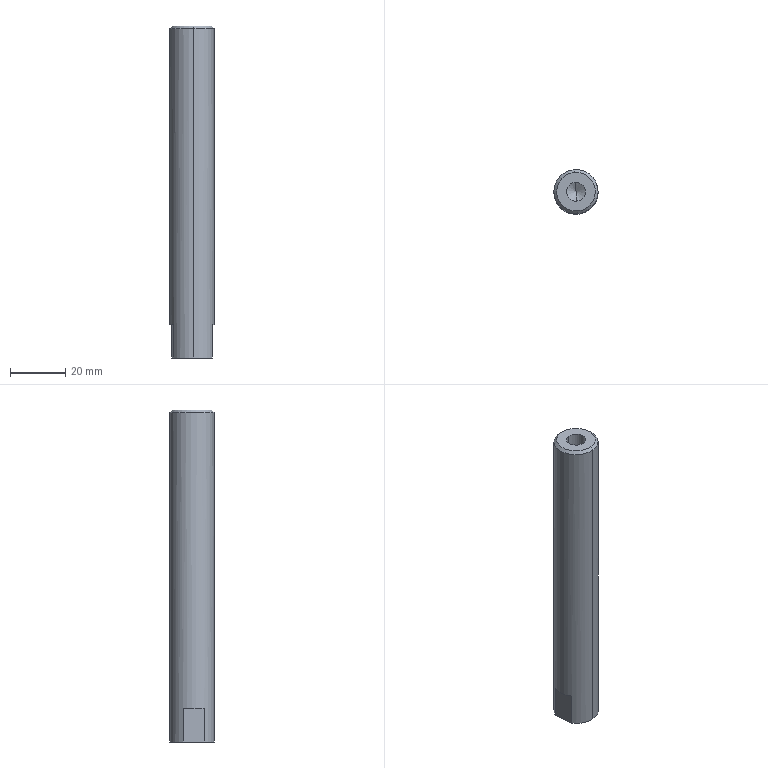Component | SolidWorks | DC-46-015-1 | 1 solid | 14 faces | box 16 x 16 x 120 mm | volume 23236 mm3 | plane 6 | cylinder 4 | cone 4 | commonest cylinder face diameters 6.8 x2 16 x2
build123d program:
from build123d import *

# Parameters (mm, degrees)
SKETCH1_R             = 8
BOSS_EXTRUDE1_DEPTH   = 60
CHAMFER1_SIZE         = 1
M8_TAPPED_HOLE1_D     = 6.8
M8_TAPPED_HOLE1_DEPTH = 19.75
M8_TAPPED_HOLE1_TIP   = 2.043
SKETCH5_W             = 7.746
SKETCH5_H             = 2
CUT_EXTRUDE1_DEPTH    = 12


with BuildPart() as part:
    # Sketch1 → Boss-Extrude1 (new, symmetric)
    with BuildSketch(Plane.XY):
        Circle(SKETCH1_R)
    extrude(amount=BOSS_EXTRUDE1_DEPTH, both=True)

    # Chamfer1
    chamfer1_edges = [part.edges().sort_by_distance(p)[0] for p in [
        (-8, 0, 60),
    ]]
    chamfer(chamfer1_edges, length=CHAMFER1_SIZE)

    # M8 Tapped Hole1
    with Locations(Plane.XY.offset(60)):
        with Locations((0, 0)):
            Hole(M8_TAPPED_HOLE1_D / 2, depth=M8_TAPPED_HOLE1_DEPTH)
            with Locations((0, 0, -(M8_TAPPED_HOLE1_DEPTH + M8_TAPPED_HOLE1_TIP / 2))):  # 118° drill point
                Cone(0, M8_TAPPED_HOLE1_D / 2, M8_TAPPED_HOLE1_TIP, mode=Mode.SUBTRACT)

    # Sketch5 → Cut-Extrude1 (cut)
    with BuildSketch(Plane(origin=(0, 0, -60), x_dir=(-1, 0, 0), z_dir=(0, 0, -1))):
        with Locations((0, -8)):
            Rectangle(SKETCH5_W, SKETCH5_H)
        with Locations((0, 8)):
            Rectangle(SKETCH5_W, SKETCH5_H)
    extrude(amount=-CUT_EXTRUDE1_DEPTH, mode=Mode.SUBTRACT)


solid = part.part

# Placed as in the assembly
solid = solid.moved(Location((264.365, 247.727, 2018.633), (0, 0, 95.045)))